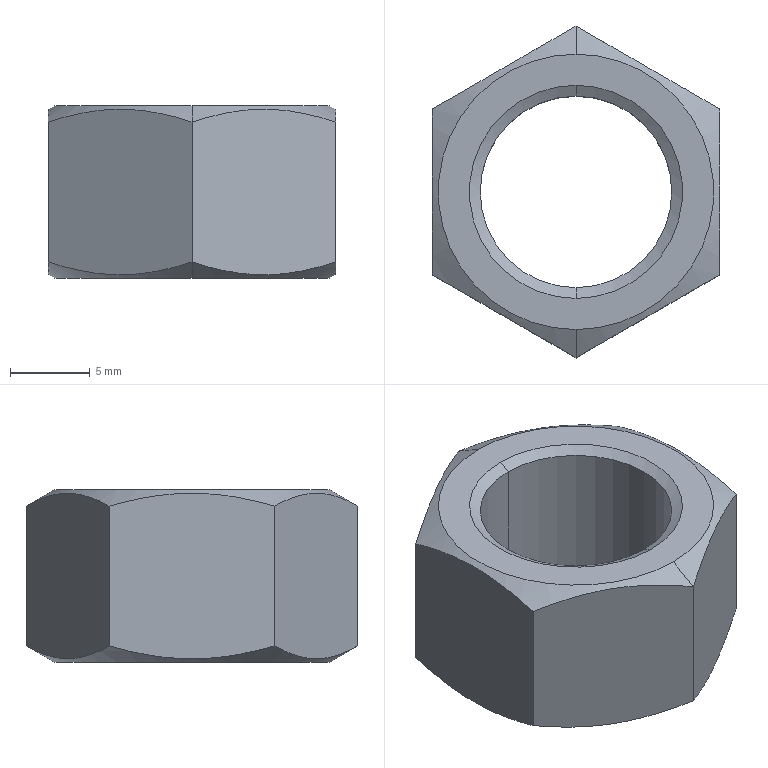Component | SolidWorks | Cylinder-1_hex nuts 1-fine pitch-grades ab gb-5 | 1 solid | 18 faces | box 18 x 20.78 x 10.8 mm | volume 1770 mm3 | cone 8 | plane 8 | cylinder 2 | commonest cylinder face diameters 12 x2
STEP:
#1=COLOUR_RGB('',0.7922,0.8196,0.9333);
#2=FILL_AREA_STYLE_COLOUR('',#1);
#3=FILL_AREA_STYLE('',(#2));
#4=SURFACE_STYLE_FILL_AREA(#3);
#5=SURFACE_SIDE_STYLE('',(#4));
#6=SURFACE_STYLE_USAGE(.BOTH.,#5);
#7=PRESENTATION_STYLE_ASSIGNMENT((#6));
#8=CARTESIAN_POINT('',(-8.211,1.906,-6.45));
#9=VERTEX_POINT('',#8);
#10=CARTESIAN_POINT('',(-8.211,2.378,-6.45));
#11=VERTEX_POINT('',#10);
#12=CARTESIAN_POINT('',(-8.211,2.142,-6.45));
#13=DIRECTION('',(-0.,0.,1.));
#14=DIRECTION('',(0.,-1.,0.));
#15=AXIS2_PLACEMENT_3D('',#12,#13,#14);
#16=CIRCLE('',#15,0.2362);
#17=EDGE_CURVE('',#9,#11,#16,.T.);
#18=ORIENTED_EDGE('',*,*,#17,.F.);
#19=CARTESIAN_POINT('',(-8.211,1.879,-6.435));
#20=VERTEX_POINT('',#19);
#21=CARTESIAN_POINT('',(-8.211,1.906,-6.45));
#22=DIRECTION('',(-0.,-0.866,0.5));
#23=VECTOR('',#22,39.37);
#24=LINE('',#21,#23);
#25=EDGE_CURVE('',#9,#20,#24,.T.);
#26=ORIENTED_EDGE('',*,*,#25,.T.);
#27=CARTESIAN_POINT('',(-8.211,2.405,-6.435));
#28=VERTEX_POINT('',#27);
#29=CARTESIAN_POINT('',(-8.211,2.142,-6.435));
#30=DIRECTION('',(0.,-0.,-1.));
#31=DIRECTION('',(0.,-1.,0.));
#32=AXIS2_PLACEMENT_3D('',#29,#30,#31);
#33=CIRCLE('',#32,0.2628);
#34=EDGE_CURVE('',#28,#20,#33,.T.);
#35=ORIENTED_EDGE('',*,*,#34,.F.);
#36=CARTESIAN_POINT('',(-8.211,2.378,-6.45));
#37=DIRECTION('',(0.,0.866,0.5));
#38=VECTOR('',#37,39.37);
#39=LINE('',#36,#38);
#40=EDGE_CURVE('',#11,#28,#39,.T.);
#41=ORIENTED_EDGE('',*,*,#40,.F.);
#42=EDGE_LOOP('',(#18,#26,#35,#41));
#43=FACE_OUTER_BOUND('',#42,.T.);
#44=CARTESIAN_POINT('',(-8.211,2.142,-6.45));
#45=DIRECTION('',(-0.,0.,1.));
#46=DIRECTION('',(0.,1.,0.));
#47=AXIS2_PLACEMENT_3D('',#44,#45,#46);
#48=CONICAL_SURFACE('',#47,0.2362,1.047);
#49=ADVANCED_FACE('',(#43),#48,.F.);
#50=CARTESIAN_POINT('',(-8.211,2.378,-6.834));
#51=VERTEX_POINT('',#50);
#52=CARTESIAN_POINT('',(-8.211,1.906,-6.834));
#53=VERTEX_POINT('',#52);
#54=CARTESIAN_POINT('',(-8.211,2.142,-6.834));
#55=DIRECTION('',(0.,-0.,-1.));
#56=DIRECTION('',(0.,-1.,0.));
#57=AXIS2_PLACEMENT_3D('',#54,#55,#56);
#58=CIRCLE('',#57,0.2362);
#59=EDGE_CURVE('',#51,#53,#58,.T.);
#60=ORIENTED_EDGE('',*,*,#59,.F.);
#61=CARTESIAN_POINT('',(-8.211,2.394,-6.86));
#62=VERTEX_POINT('',#61);
#63=CARTESIAN_POINT('',(-8.211,2.394,-6.86));
#64=DIRECTION('',(-0.,0.5,-0.866));
#65=VECTOR('',#64,39.37);
#66=LINE('',#63,#65);
#67=EDGE_CURVE('',#51,#62,#66,.T.);
#68=ORIENTED_EDGE('',*,*,#67,.T.);
#69=CARTESIAN_POINT('',(-8.211,1.891,-6.86));
#70=VERTEX_POINT('',#69);
#71=CARTESIAN_POINT('',(-8.211,2.142,-6.86));
#72=DIRECTION('',(-0.,0.,1.));
#73=DIRECTION('',(0.,-1.,0.));
#74=AXIS2_PLACEMENT_3D('',#71,#72,#73);
#75=CIRCLE('',#74,0.2516);
#76=EDGE_CURVE('',#70,#62,#75,.T.);
#77=ORIENTED_EDGE('',*,*,#76,.F.);
#78=CARTESIAN_POINT('',(-8.211,1.891,-6.86));
#79=DIRECTION('',(-0.,-0.5,-0.866));
#80=VECTOR('',#79,39.37);
#81=LINE('',#78,#80);
#82=EDGE_CURVE('',#53,#70,#81,.T.);
#83=ORIENTED_EDGE('',*,*,#82,.F.);
#84=EDGE_LOOP('',(#60,#68,#77,#83));
#85=FACE_OUTER_BOUND('',#84,.T.);
#86=CARTESIAN_POINT('',(-8.211,2.142,-6.86));
#87=DIRECTION('',(0.,-0.,-1.));
#88=DIRECTION('',(0.,-1.,0.));
#89=AXIS2_PLACEMENT_3D('',#86,#87,#88);
#90=CONICAL_SURFACE('',#89,0.2516,0.5236);
#91=ADVANCED_FACE('',(#85),#90,.F.);
#92=CARTESIAN_POINT('',(-8.211,1.803,-6.435));
#93=VERTEX_POINT('',#92);
#94=CARTESIAN_POINT('',(-8.211,2.482,-6.435));
#95=VERTEX_POINT('',#94);
#96=CARTESIAN_POINT('',(-8.211,2.142,-6.435));
#97=DIRECTION('',(0.,-0.,-1.));
#98=DIRECTION('',(0.,-1.,0.));
#99=AXIS2_PLACEMENT_3D('',#96,#97,#98);
#100=CIRCLE('',#99,0.3396);
#101=EDGE_CURVE('',#93,#95,#100,.T.);
#102=ORIENTED_EDGE('',*,*,#101,.T.);
#103=CARTESIAN_POINT('',(-8.211,2.551,-6.475));
#104=VERTEX_POINT('',#103);
#105=CARTESIAN_POINT('',(-8.211,2.482,-6.435));
#106=DIRECTION('',(-0.,0.866,-0.5));
#107=VECTOR('',#106,39.37);
#108=LINE('',#105,#107);
#109=EDGE_CURVE('',#95,#104,#108,.T.);
#110=ORIENTED_EDGE('',*,*,#109,.T.);
#111=CARTESIAN_POINT('',(-8.565,2.347,-6.475));
#112=VERTEX_POINT('',#111);
#113=CARTESIAN_POINT('',(-8.211,2.551,-6.475));
#114=CARTESIAN_POINT('',(-8.24,2.535,-6.466));
#115=CARTESIAN_POINT('',(-8.269,2.518,-6.458));
#116=CARTESIAN_POINT('',(-8.328,2.484,-6.447));
#117=CARTESIAN_POINT('',(-8.358,2.467,-6.444));
#118=CARTESIAN_POINT('',(-8.403,2.441,-6.444));
#119=CARTESIAN_POINT('',(-8.418,2.432,-6.444));
#120=CARTESIAN_POINT('',(-8.448,2.415,-6.447));
#121=CARTESIAN_POINT('',(-8.463,2.406,-6.449));
#122=CARTESIAN_POINT('',(-8.507,2.38,-6.458));
#123=CARTESIAN_POINT('',(-8.536,2.363,-6.466));
#124=CARTESIAN_POINT('',(-8.565,2.347,-6.475));
#125=B_SPLINE_CURVE_WITH_KNOTS('',3,(#113,#114,#115,#116,#117,#118,#119,#120,#121,#122,#123,#124),.UNSPECIFIED.,.F.,.F.,(4,2,2,2,2,4),(0.00000024,0.002624,0.005248,0.00656,0.007872,0.0105),.UNSPECIFIED.);
#126=EDGE_CURVE('',#104,#112,#125,.T.);
#127=ORIENTED_EDGE('',*,*,#126,.T.);
#128=CARTESIAN_POINT('',(-8.565,1.938,-6.475));
#129=VERTEX_POINT('',#128);
#130=CARTESIAN_POINT('',(-8.565,2.347,-6.475));
#131=CARTESIAN_POINT('',(-8.565,2.314,-6.466));
#132=CARTESIAN_POINT('',(-8.565,2.28,-6.458));
#133=CARTESIAN_POINT('',(-8.565,2.229,-6.449));
#134=CARTESIAN_POINT('',(-8.565,2.212,-6.447));
#135=CARTESIAN_POINT('',(-8.565,2.177,-6.444));
#136=CARTESIAN_POINT('',(-8.565,2.16,-6.444));
#137=CARTESIAN_POINT('',(-8.565,2.108,-6.444));
#138=CARTESIAN_POINT('',(-8.565,2.073,-6.447));
#139=CARTESIAN_POINT('',(-8.565,2.005,-6.458));
#140=CARTESIAN_POINT('',(-8.565,1.971,-6.466));
#141=CARTESIAN_POINT('',(-8.565,1.938,-6.475));
#142=B_SPLINE_CURVE_WITH_KNOTS('',3,(#130,#131,#132,#133,#134,#135,#136,#137,#138,#139,#140,#141),.UNSPECIFIED.,.F.,.F.,(4,2,2,2,2,4),(0.003845,0.006467,0.007778,0.009089,0.01171,0.01433),.UNSPECIFIED.);
#143=EDGE_CURVE('',#112,#129,#142,.T.);
#144=ORIENTED_EDGE('',*,*,#143,.T.);
#145=CARTESIAN_POINT('',(-8.211,1.733,-6.475));
#146=VERTEX_POINT('',#145);
#147=CARTESIAN_POINT('',(-8.565,1.938,-6.475));
#148=CARTESIAN_POINT('',(-8.536,1.921,-6.466));
#149=CARTESIAN_POINT('',(-8.507,1.904,-6.458));
#150=CARTESIAN_POINT('',(-8.448,1.87,-6.447));
#151=CARTESIAN_POINT('',(-8.419,1.853,-6.444));
#152=CARTESIAN_POINT('',(-8.373,1.827,-6.444));
#153=CARTESIAN_POINT('',(-8.358,1.818,-6.444));
#154=CARTESIAN_POINT('',(-8.328,1.801,-6.447));
#155=CARTESIAN_POINT('',(-8.313,1.792,-6.449));
#156=CARTESIAN_POINT('',(-8.269,1.767,-6.458));
#157=CARTESIAN_POINT('',(-8.24,1.75,-6.466));
#158=CARTESIAN_POINT('',(-8.211,1.733,-6.475));
#159=B_SPLINE_CURVE_WITH_KNOTS('',3,(#147,#148,#149,#150,#151,#152,#153,#154,#155,#156,#157,#158),.UNSPECIFIED.,.F.,.F.,(4,2,2,2,2,4),(0.00000024,0.002624,0.005248,0.00656,0.007872,0.0105),.UNSPECIFIED.);
#160=EDGE_CURVE('',#129,#146,#159,.T.);
#161=ORIENTED_EDGE('',*,*,#160,.T.);
#162=CARTESIAN_POINT('',(-8.211,1.803,-6.435));
#163=DIRECTION('',(-0.,-0.866,-0.5));
#164=VECTOR('',#163,39.37);
#165=LINE('',#162,#164);
#166=EDGE_CURVE('',#93,#146,#165,.T.);
#167=ORIENTED_EDGE('',*,*,#166,.F.);
#168=EDGE_LOOP('',(#102,#110,#127,#144,#161,#167));
#169=FACE_OUTER_BOUND('',#168,.T.);
#170=CARTESIAN_POINT('',(-8.211,2.142,-6.435));
#171=DIRECTION('',(0.,-0.,-1.));
#172=DIRECTION('',(0.,-1.,0.));
#173=AXIS2_PLACEMENT_3D('',#170,#171,#172);
#174=CONICAL_SURFACE('',#173,0.3396,1.047);
#175=ADVANCED_FACE('',(#169),#174,.T.);
#176=CARTESIAN_POINT('',(-8.211,1.803,-6.86));
#177=VERTEX_POINT('',#176);
#178=CARTESIAN_POINT('',(-8.211,2.482,-6.86));
#179=VERTEX_POINT('',#178);
#180=CARTESIAN_POINT('',(-8.211,2.142,-6.86));
#181=DIRECTION('',(0.,-0.,-1.));
#182=DIRECTION('',(0.,-1.,0.));
#183=AXIS2_PLACEMENT_3D('',#180,#181,#182);
#184=CIRCLE('',#183,0.3396);
#185=EDGE_CURVE('',#177,#179,#184,.T.);
#186=ORIENTED_EDGE('',*,*,#185,.F.);
#187=CARTESIAN_POINT('',(-8.211,1.733,-6.82));
#188=VERTEX_POINT('',#187);
#189=CARTESIAN_POINT('',(-8.211,1.733,-6.82));
#190=DIRECTION('',(-0.,-0.866,0.5));
#191=VECTOR('',#190,39.37);
#192=LINE('',#189,#191);
#193=EDGE_CURVE('',#177,#188,#192,.T.);
#194=ORIENTED_EDGE('',*,*,#193,.T.);
#195=CARTESIAN_POINT('',(-8.565,1.938,-6.82));
#196=VERTEX_POINT('',#195);
#197=CARTESIAN_POINT('',(-8.211,1.733,-6.82));
#198=CARTESIAN_POINT('',(-8.24,1.75,-6.83));
#199=CARTESIAN_POINT('',(-8.269,1.767,-6.838));
#200=CARTESIAN_POINT('',(-8.328,1.801,-6.849));
#201=CARTESIAN_POINT('',(-8.358,1.818,-6.852));
#202=CARTESIAN_POINT('',(-8.403,1.844,-6.852));
#203=CARTESIAN_POINT('',(-8.418,1.853,-6.851));
#204=CARTESIAN_POINT('',(-8.448,1.87,-6.848));
#205=CARTESIAN_POINT('',(-8.463,1.878,-6.846));
#206=CARTESIAN_POINT('',(-8.507,1.904,-6.838));
#207=CARTESIAN_POINT('',(-8.536,1.921,-6.83));
#208=CARTESIAN_POINT('',(-8.565,1.938,-6.82));
#209=B_SPLINE_CURVE_WITH_KNOTS('',3,(#197,#198,#199,#200,#201,#202,#203,#204,#205,#206,#207,#208),.UNSPECIFIED.,.F.,.F.,(4,2,2,2,2,4),(0.00000024,0.002624,0.005248,0.00656,0.007872,0.0105),.UNSPECIFIED.);
#210=EDGE_CURVE('',#188,#196,#209,.T.);
#211=ORIENTED_EDGE('',*,*,#210,.T.);
#212=CARTESIAN_POINT('',(-8.565,2.347,-6.82));
#213=VERTEX_POINT('',#212);
#214=CARTESIAN_POINT('',(-8.565,1.938,-6.82));
#215=CARTESIAN_POINT('',(-8.565,1.971,-6.83));
#216=CARTESIAN_POINT('',(-8.565,2.005,-6.838));
#217=CARTESIAN_POINT('',(-8.565,2.073,-6.849));
#218=CARTESIAN_POINT('',(-8.565,2.108,-6.852));
#219=CARTESIAN_POINT('',(-8.565,2.16,-6.852));
#220=CARTESIAN_POINT('',(-8.565,2.177,-6.851));
#221=CARTESIAN_POINT('',(-8.565,2.212,-6.848));
#222=CARTESIAN_POINT('',(-8.565,2.229,-6.846));
#223=CARTESIAN_POINT('',(-8.565,2.28,-6.838));
#224=CARTESIAN_POINT('',(-8.565,2.314,-6.83));
#225=CARTESIAN_POINT('',(-8.565,2.347,-6.82));
#226=B_SPLINE_CURVE_WITH_KNOTS('',3,(#214,#215,#216,#217,#218,#219,#220,#221,#222,#223,#224,#225),.UNSPECIFIED.,.F.,.F.,(4,2,2,2,2,4),(0.009237,0.01187,0.0145,0.01581,0.01712,0.01975),.UNSPECIFIED.);
#227=EDGE_CURVE('',#196,#213,#226,.T.);
#228=ORIENTED_EDGE('',*,*,#227,.T.);
#229=CARTESIAN_POINT('',(-8.211,2.551,-6.82));
#230=VERTEX_POINT('',#229);
#231=CARTESIAN_POINT('',(-8.565,2.347,-6.82));
#232=CARTESIAN_POINT('',(-8.536,2.363,-6.83));
#233=CARTESIAN_POINT('',(-8.507,2.38,-6.838));
#234=CARTESIAN_POINT('',(-8.448,2.414,-6.849));
#235=CARTESIAN_POINT('',(-8.419,2.431,-6.852));
#236=CARTESIAN_POINT('',(-8.373,2.458,-6.852));
#237=CARTESIAN_POINT('',(-8.358,2.466,-6.851));
#238=CARTESIAN_POINT('',(-8.328,2.484,-6.848));
#239=CARTESIAN_POINT('',(-8.313,2.492,-6.846));
#240=CARTESIAN_POINT('',(-8.269,2.518,-6.838));
#241=CARTESIAN_POINT('',(-8.24,2.535,-6.83));
#242=CARTESIAN_POINT('',(-8.211,2.551,-6.82));
#243=B_SPLINE_CURVE_WITH_KNOTS('',3,(#231,#232,#233,#234,#235,#236,#237,#238,#239,#240,#241,#242),.UNSPECIFIED.,.F.,.F.,(4,2,2,2,2,4),(0.00000024,0.002624,0.005248,0.00656,0.007872,0.0105),.UNSPECIFIED.);
#244=EDGE_CURVE('',#213,#230,#243,.T.);
#245=ORIENTED_EDGE('',*,*,#244,.T.);
#246=CARTESIAN_POINT('',(-8.211,2.551,-6.82));
#247=DIRECTION('',(0.,0.866,0.5));
#248=VECTOR('',#247,39.37);
#249=LINE('',#246,#248);
#250=EDGE_CURVE('',#179,#230,#249,.T.);
#251=ORIENTED_EDGE('',*,*,#250,.F.);
#252=EDGE_LOOP('',(#186,#194,#211,#228,#245,#251));
#253=FACE_OUTER_BOUND('',#252,.T.);
#254=CARTESIAN_POINT('',(-8.211,2.142,-6.82));
#255=DIRECTION('',(-0.,0.,1.));
#256=DIRECTION('',(0.,1.,0.));
#257=AXIS2_PLACEMENT_3D('',#254,#255,#256);
#258=CONICAL_SURFACE('',#257,0.4091,1.047);
#259=ADVANCED_FACE('',(#253),#258,.T.);
#260=ORIENTED_EDGE('',*,*,#59,.T.);
#261=CARTESIAN_POINT('',(-8.211,1.906,-6.86));
#262=DIRECTION('',(-0.,0.,1.));
#263=VECTOR('',#262,39.37);
#264=LINE('',#261,#263);
#265=EDGE_CURVE('',#53,#9,#264,.T.);
#266=ORIENTED_EDGE('',*,*,#265,.T.);
#267=ORIENTED_EDGE('',*,*,#17,.T.);
#268=CARTESIAN_POINT('',(-8.211,2.378,-6.86));
#269=DIRECTION('',(-0.,0.,1.));
#270=VECTOR('',#269,39.37);
#271=LINE('',#268,#270);
#272=EDGE_CURVE('',#51,#11,#271,.T.);
#273=ORIENTED_EDGE('',*,*,#272,.F.);
#274=EDGE_LOOP('',(#260,#266,#267,#273));
#275=FACE_OUTER_BOUND('',#274,.T.);
#276=CARTESIAN_POINT('',(-8.211,2.142,-6.86));
#277=DIRECTION('',(-0.,0.,1.));
#278=DIRECTION('',(0.,1.,0.));
#279=AXIS2_PLACEMENT_3D('',#276,#277,#278);
#280=CYLINDRICAL_SURFACE('',#279,0.2362);
#281=ADVANCED_FACE('',(#275),#280,.F.);
#282=CARTESIAN_POINT('',(-7.857,1.938,-6.475));
#283=VERTEX_POINT('',#282);
#284=CARTESIAN_POINT('',(-7.857,2.347,-6.475));
#285=VERTEX_POINT('',#284);
#286=CARTESIAN_POINT('',(-7.857,1.938,-6.475));
#287=CARTESIAN_POINT('',(-7.857,1.971,-6.466));
#288=CARTESIAN_POINT('',(-7.857,2.005,-6.458));
#289=CARTESIAN_POINT('',(-7.857,2.073,-6.447));
#290=CARTESIAN_POINT('',(-7.857,2.108,-6.444));
#291=CARTESIAN_POINT('',(-7.857,2.16,-6.444));
#292=CARTESIAN_POINT('',(-7.857,2.177,-6.444));
#293=CARTESIAN_POINT('',(-7.857,2.212,-6.447));
#294=CARTESIAN_POINT('',(-7.857,2.229,-6.449));
#295=CARTESIAN_POINT('',(-7.857,2.28,-6.458));
#296=CARTESIAN_POINT('',(-7.857,2.314,-6.466));
#297=CARTESIAN_POINT('',(-7.857,2.347,-6.475));
#298=B_SPLINE_CURVE_WITH_KNOTS('',3,(#286,#287,#288,#289,#290,#291,#292,#293,#294,#295,#296,#297),.UNSPECIFIED.,.F.,.F.,(4,2,2,2,2,4),(0.009237,0.01187,0.0145,0.01581,0.01712,0.01975),.UNSPECIFIED.);
#299=EDGE_CURVE('',#283,#285,#298,.T.);
#300=ORIENTED_EDGE('',*,*,#299,.F.);
#301=CARTESIAN_POINT('',(-7.857,1.938,-6.82));
#302=VERTEX_POINT('',#301);
#303=CARTESIAN_POINT('',(-7.857,1.938,-6.86));
#304=DIRECTION('',(-0.,0.,1.));
#305=VECTOR('',#304,39.37);
#306=LINE('',#303,#305);
#307=EDGE_CURVE('',#302,#283,#306,.T.);
#308=ORIENTED_EDGE('',*,*,#307,.F.);
#309=CARTESIAN_POINT('',(-7.857,2.347,-6.82));
#310=VERTEX_POINT('',#309);
#311=CARTESIAN_POINT('',(-7.857,2.347,-6.82));
#312=CARTESIAN_POINT('',(-7.857,2.314,-6.83));
#313=CARTESIAN_POINT('',(-7.857,2.28,-6.838));
#314=CARTESIAN_POINT('',(-7.857,2.229,-6.846));
#315=CARTESIAN_POINT('',(-7.857,2.212,-6.848));
#316=CARTESIAN_POINT('',(-7.857,2.177,-6.851));
#317=CARTESIAN_POINT('',(-7.857,2.16,-6.852));
#318=CARTESIAN_POINT('',(-7.857,2.108,-6.852));
#319=CARTESIAN_POINT('',(-7.857,2.073,-6.849));
#320=CARTESIAN_POINT('',(-7.857,2.005,-6.838));
#321=CARTESIAN_POINT('',(-7.857,1.971,-6.83));
#322=CARTESIAN_POINT('',(-7.857,1.938,-6.82));
#323=B_SPLINE_CURVE_WITH_KNOTS('',3,(#311,#312,#313,#314,#315,#316,#317,#318,#319,#320,#321,#322),.UNSPECIFIED.,.F.,.F.,(4,2,2,2,2,4),(0.003845,0.006467,0.007778,0.009089,0.01171,0.01433),.UNSPECIFIED.);
#324=EDGE_CURVE('',#310,#302,#323,.T.);
#325=ORIENTED_EDGE('',*,*,#324,.F.);
#326=CARTESIAN_POINT('',(-7.857,2.347,-6.86));
#327=DIRECTION('',(-0.,0.,1.));
#328=VECTOR('',#327,39.37);
#329=LINE('',#326,#328);
#330=EDGE_CURVE('',#310,#285,#329,.T.);
#331=ORIENTED_EDGE('',*,*,#330,.T.);
#332=EDGE_LOOP('',(#300,#308,#325,#331));
#333=FACE_OUTER_BOUND('',#332,.T.);
#334=CARTESIAN_POINT('',(-7.857,1.938,-6.86));
#335=DIRECTION('',(1.,-0.,0.));
#336=DIRECTION('',(0.,-0.,-1.));
#337=AXIS2_PLACEMENT_3D('',#334,#335,#336);
#338=PLANE('',#337);
#339=ADVANCED_FACE('',(#333),#338,.T.);
#340=CARTESIAN_POINT('',(-8.211,1.733,-6.475));
#341=CARTESIAN_POINT('',(-8.182,1.75,-6.466));
#342=CARTESIAN_POINT('',(-8.153,1.767,-6.458));
#343=CARTESIAN_POINT('',(-8.094,1.801,-6.447));
#344=CARTESIAN_POINT('',(-8.064,1.818,-6.444));
#345=CARTESIAN_POINT('',(-8.019,1.844,-6.444));
#346=CARTESIAN_POINT('',(-8.004,1.853,-6.444));
#347=CARTESIAN_POINT('',(-7.974,1.87,-6.447));
#348=CARTESIAN_POINT('',(-7.959,1.878,-6.449));
#349=CARTESIAN_POINT('',(-7.915,1.904,-6.458));
#350=CARTESIAN_POINT('',(-7.886,1.921,-6.466));
#351=CARTESIAN_POINT('',(-7.857,1.938,-6.475));
#352=B_SPLINE_CURVE_WITH_KNOTS('',3,(#340,#341,#342,#343,#344,#345,#346,#347,#348,#349,#350,#351),.UNSPECIFIED.,.F.,.F.,(4,2,2,2,2,4),(0.00000024,0.002624,0.005248,0.00656,0.007872,0.0105),.UNSPECIFIED.);
#353=EDGE_CURVE('',#146,#283,#352,.T.);
#354=ORIENTED_EDGE('',*,*,#353,.F.);
#355=CARTESIAN_POINT('',(-8.211,1.733,-6.86));
#356=DIRECTION('',(-0.,0.,1.));
#357=VECTOR('',#356,39.37);
#358=LINE('',#355,#357);
#359=EDGE_CURVE('',#188,#146,#358,.T.);
#360=ORIENTED_EDGE('',*,*,#359,.F.);
#361=CARTESIAN_POINT('',(-7.857,1.938,-6.82));
#362=CARTESIAN_POINT('',(-7.885,1.921,-6.83));
#363=CARTESIAN_POINT('',(-7.915,1.904,-6.838));
#364=CARTESIAN_POINT('',(-7.974,1.87,-6.849));
#365=CARTESIAN_POINT('',(-8.003,1.853,-6.852));
#366=CARTESIAN_POINT('',(-8.048,1.827,-6.852));
#367=CARTESIAN_POINT('',(-8.064,1.818,-6.851));
#368=CARTESIAN_POINT('',(-8.094,1.801,-6.848));
#369=CARTESIAN_POINT('',(-8.108,1.792,-6.846));
#370=CARTESIAN_POINT('',(-8.153,1.767,-6.838));
#371=CARTESIAN_POINT('',(-8.182,1.75,-6.83));
#372=CARTESIAN_POINT('',(-8.211,1.733,-6.82));
#373=B_SPLINE_CURVE_WITH_KNOTS('',3,(#361,#362,#363,#364,#365,#366,#367,#368,#369,#370,#371,#372),.UNSPECIFIED.,.F.,.F.,(4,2,2,2,2,4),(0.00000024,0.002624,0.005248,0.00656,0.007872,0.0105),.UNSPECIFIED.);
#374=EDGE_CURVE('',#302,#188,#373,.T.);
#375=ORIENTED_EDGE('',*,*,#374,.F.);
#376=ORIENTED_EDGE('',*,*,#307,.T.);
#377=EDGE_LOOP('',(#354,#360,#375,#376));
#378=FACE_OUTER_BOUND('',#377,.T.);
#379=CARTESIAN_POINT('',(-8.211,1.733,-6.86));
#380=DIRECTION('',(0.5,-0.866,0.));
#381=DIRECTION('',(0.866,0.5,-0.));
#382=AXIS2_PLACEMENT_3D('',#379,#380,#381);
#383=PLANE('',#382);
#384=ADVANCED_FACE('',(#378),#383,.T.);
#385=ORIENTED_EDGE('',*,*,#160,.F.);
#386=CARTESIAN_POINT('',(-8.565,1.938,-6.86));
#387=DIRECTION('',(-0.,0.,1.));
#388=VECTOR('',#387,39.37);
#389=LINE('',#386,#388);
#390=EDGE_CURVE('',#196,#129,#389,.T.);
#391=ORIENTED_EDGE('',*,*,#390,.F.);
#392=ORIENTED_EDGE('',*,*,#210,.F.);
#393=ORIENTED_EDGE('',*,*,#359,.T.);
#394=EDGE_LOOP('',(#385,#391,#392,#393));
#395=FACE_OUTER_BOUND('',#394,.T.);
#396=CARTESIAN_POINT('',(-8.565,1.938,-6.86));
#397=DIRECTION('',(-0.5,-0.866,0.));
#398=DIRECTION('',(0.866,-0.5,0.));
#399=AXIS2_PLACEMENT_3D('',#396,#397,#398);
#400=PLANE('',#399);
#401=ADVANCED_FACE('',(#395),#400,.T.);
#402=ORIENTED_EDGE('',*,*,#143,.F.);
#403=CARTESIAN_POINT('',(-8.565,2.347,-6.86));
#404=DIRECTION('',(-0.,0.,1.));
#405=VECTOR('',#404,39.37);
#406=LINE('',#403,#405);
#407=EDGE_CURVE('',#213,#112,#406,.T.);
#408=ORIENTED_EDGE('',*,*,#407,.F.);
#409=ORIENTED_EDGE('',*,*,#227,.F.);
#410=ORIENTED_EDGE('',*,*,#390,.T.);
#411=EDGE_LOOP('',(#402,#408,#409,#410));
#412=FACE_OUTER_BOUND('',#411,.T.);
#413=CARTESIAN_POINT('',(-8.565,2.347,-6.86));
#414=DIRECTION('',(-1.,0.,-0.));
#415=DIRECTION('',(-0.,-1.,0.));
#416=AXIS2_PLACEMENT_3D('',#413,#414,#415);
#417=PLANE('',#416);
#418=ADVANCED_FACE('',(#412),#417,.T.);
#419=ORIENTED_EDGE('',*,*,#126,.F.);
#420=CARTESIAN_POINT('',(-8.211,2.551,-6.86));
#421=DIRECTION('',(-0.,0.,1.));
#422=VECTOR('',#421,39.37);
#423=LINE('',#420,#422);
#424=EDGE_CURVE('',#230,#104,#423,.T.);
#425=ORIENTED_EDGE('',*,*,#424,.F.);
#426=ORIENTED_EDGE('',*,*,#244,.F.);
#427=ORIENTED_EDGE('',*,*,#407,.T.);
#428=EDGE_LOOP('',(#419,#425,#426,#427));
#429=FACE_OUTER_BOUND('',#428,.T.);
#430=CARTESIAN_POINT('',(-8.211,2.551,-6.86));
#431=DIRECTION('',(-0.5,0.866,-0.));
#432=DIRECTION('',(-0.866,-0.5,0.));
#433=AXIS2_PLACEMENT_3D('',#430,#431,#432);
#434=PLANE('',#433);
#435=ADVANCED_FACE('',(#429),#434,.T.);
#436=CARTESIAN_POINT('',(-7.857,2.347,-6.475));
#437=CARTESIAN_POINT('',(-7.885,2.363,-6.466));
#438=CARTESIAN_POINT('',(-7.915,2.38,-6.458));
#439=CARTESIAN_POINT('',(-7.974,2.414,-6.447));
#440=CARTESIAN_POINT('',(-8.003,2.431,-6.444));
#441=CARTESIAN_POINT('',(-8.048,2.458,-6.444));
#442=CARTESIAN_POINT('',(-8.064,2.466,-6.444));
#443=CARTESIAN_POINT('',(-8.094,2.484,-6.447));
#444=CARTESIAN_POINT('',(-8.108,2.492,-6.449));
#445=CARTESIAN_POINT('',(-8.153,2.518,-6.458));
#446=CARTESIAN_POINT('',(-8.182,2.535,-6.466));
#447=CARTESIAN_POINT('',(-8.211,2.551,-6.475));
#448=B_SPLINE_CURVE_WITH_KNOTS('',3,(#436,#437,#438,#439,#440,#441,#442,#443,#444,#445,#446,#447),.UNSPECIFIED.,.F.,.F.,(4,2,2,2,2,4),(0.00000024,0.002624,0.005248,0.00656,0.007872,0.0105),.UNSPECIFIED.);
#449=EDGE_CURVE('',#285,#104,#448,.T.);
#450=ORIENTED_EDGE('',*,*,#449,.F.);
#451=ORIENTED_EDGE('',*,*,#330,.F.);
#452=CARTESIAN_POINT('',(-8.211,2.551,-6.82));
#453=CARTESIAN_POINT('',(-8.182,2.535,-6.83));
#454=CARTESIAN_POINT('',(-8.153,2.518,-6.838));
#455=CARTESIAN_POINT('',(-8.094,2.484,-6.849));
#456=CARTESIAN_POINT('',(-8.064,2.467,-6.852));
#457=CARTESIAN_POINT('',(-8.019,2.441,-6.852));
#458=CARTESIAN_POINT('',(-8.004,2.432,-6.851));
#459=CARTESIAN_POINT('',(-7.974,2.415,-6.848));
#460=CARTESIAN_POINT('',(-7.959,2.406,-6.846));
#461=CARTESIAN_POINT('',(-7.915,2.38,-6.838));
#462=CARTESIAN_POINT('',(-7.886,2.363,-6.83));
#463=CARTESIAN_POINT('',(-7.857,2.347,-6.82));
#464=B_SPLINE_CURVE_WITH_KNOTS('',3,(#452,#453,#454,#455,#456,#457,#458,#459,#460,#461,#462,#463),.UNSPECIFIED.,.F.,.F.,(4,2,2,2,2,4),(0.00000024,0.002624,0.005248,0.00656,0.007872,0.0105),.UNSPECIFIED.);
#465=EDGE_CURVE('',#230,#310,#464,.T.);
#466=ORIENTED_EDGE('',*,*,#465,.F.);
#467=ORIENTED_EDGE('',*,*,#424,.T.);
#468=EDGE_LOOP('',(#450,#451,#466,#467));
#469=FACE_OUTER_BOUND('',#468,.T.);
#470=CARTESIAN_POINT('',(-7.857,2.347,-6.86));
#471=DIRECTION('',(0.5,0.866,-0.));
#472=DIRECTION('',(-0.866,0.5,-0.));
#473=AXIS2_PLACEMENT_3D('',#470,#471,#472);
#474=PLANE('',#473);
#475=ADVANCED_FACE('',(#469),#474,.T.);
#476=ORIENTED_EDGE('',*,*,#76,.T.);
#477=CARTESIAN_POINT('',(-8.211,2.142,-6.86));
#478=DIRECTION('',(-0.,0.,1.));
#479=DIRECTION('',(0.,-1.,0.));
#480=AXIS2_PLACEMENT_3D('',#477,#478,#479);
#481=CIRCLE('',#480,0.2516);
#482=EDGE_CURVE('',#62,#70,#481,.T.);
#483=ORIENTED_EDGE('',*,*,#482,.T.);
#484=EDGE_LOOP('',(#476,#483));
#485=FACE_BOUND('',#484,.T.);
#486=CARTESIAN_POINT('',(-8.211,2.142,-6.86));
#487=DIRECTION('',(0.,-0.,-1.));
#488=DIRECTION('',(0.,-1.,0.));
#489=AXIS2_PLACEMENT_3D('',#486,#487,#488);
#490=CIRCLE('',#489,0.3396);
#491=EDGE_CURVE('',#179,#177,#490,.T.);
#492=ORIENTED_EDGE('',*,*,#491,.T.);
#493=ORIENTED_EDGE('',*,*,#185,.T.);
#494=EDGE_LOOP('',(#492,#493));
#495=FACE_OUTER_BOUND('',#494,.T.);
#496=CARTESIAN_POINT('',(-7.857,1.528,-6.86));
#497=DIRECTION('',(0.,-0.,-1.));
#498=DIRECTION('',(-0.,-1.,0.));
#499=AXIS2_PLACEMENT_3D('',#496,#497,#498);
#500=PLANE('',#499);
#501=ADVANCED_FACE('',(#485,#495),#500,.T.);
#502=ORIENTED_EDGE('',*,*,#34,.T.);
#503=CARTESIAN_POINT('',(-8.211,2.142,-6.435));
#504=DIRECTION('',(0.,-0.,-1.));
#505=DIRECTION('',(0.,-1.,0.));
#506=AXIS2_PLACEMENT_3D('',#503,#504,#505);
#507=CIRCLE('',#506,0.2628);
#508=EDGE_CURVE('',#20,#28,#507,.T.);
#509=ORIENTED_EDGE('',*,*,#508,.T.);
#510=EDGE_LOOP('',(#502,#509));
#511=FACE_BOUND('',#510,.T.);
#512=ORIENTED_EDGE('',*,*,#101,.F.);
#513=CARTESIAN_POINT('',(-8.211,2.142,-6.435));
#514=DIRECTION('',(0.,-0.,-1.));
#515=DIRECTION('',(0.,-1.,0.));
#516=AXIS2_PLACEMENT_3D('',#513,#514,#515);
#517=CIRCLE('',#516,0.3396);
#518=EDGE_CURVE('',#95,#93,#517,.T.);
#519=ORIENTED_EDGE('',*,*,#518,.F.);
#520=EDGE_LOOP('',(#512,#519));
#521=FACE_OUTER_BOUND('',#520,.T.);
#522=CARTESIAN_POINT('',(-7.857,1.528,-6.435));
#523=DIRECTION('',(0.,-0.,-1.));
#524=DIRECTION('',(-0.,-1.,0.));
#525=AXIS2_PLACEMENT_3D('',#522,#523,#524);
#526=PLANE('',#525);
#527=ADVANCED_FACE('',(#511,#521),#526,.F.);
#528=ORIENTED_EDGE('',*,*,#265,.F.);
#529=CARTESIAN_POINT('',(-8.211,2.142,-6.834));
#530=DIRECTION('',(0.,-0.,-1.));
#531=DIRECTION('',(0.,-1.,0.));
#532=AXIS2_PLACEMENT_3D('',#529,#530,#531);
#533=CIRCLE('',#532,0.2362);
#534=EDGE_CURVE('',#53,#51,#533,.T.);
#535=ORIENTED_EDGE('',*,*,#534,.T.);
#536=ORIENTED_EDGE('',*,*,#272,.T.);
#537=CARTESIAN_POINT('',(-8.211,2.142,-6.45));
#538=DIRECTION('',(-0.,0.,1.));
#539=DIRECTION('',(0.,-1.,0.));
#540=AXIS2_PLACEMENT_3D('',#537,#538,#539);
#541=CIRCLE('',#540,0.2362);
#542=EDGE_CURVE('',#11,#9,#541,.T.);
#543=ORIENTED_EDGE('',*,*,#542,.T.);
#544=EDGE_LOOP('',(#528,#535,#536,#543));
#545=FACE_OUTER_BOUND('',#544,.T.);
#546=CARTESIAN_POINT('',(-8.211,2.142,-6.86));
#547=DIRECTION('',(-0.,0.,1.));
#548=DIRECTION('',(0.,1.,0.));
#549=AXIS2_PLACEMENT_3D('',#546,#547,#548);
#550=CYLINDRICAL_SURFACE('',#549,0.2362);
#551=ADVANCED_FACE('',(#545),#550,.F.);
#552=ORIENTED_EDGE('',*,*,#193,.F.);
#553=ORIENTED_EDGE('',*,*,#491,.F.);
#554=ORIENTED_EDGE('',*,*,#250,.T.);
#555=ORIENTED_EDGE('',*,*,#465,.T.);
#556=ORIENTED_EDGE('',*,*,#324,.T.);
#557=ORIENTED_EDGE('',*,*,#374,.T.);
#558=EDGE_LOOP('',(#552,#553,#554,#555,#556,#557));
#559=FACE_OUTER_BOUND('',#558,.T.);
#560=CARTESIAN_POINT('',(-8.211,2.142,-6.82));
#561=DIRECTION('',(-0.,0.,1.));
#562=DIRECTION('',(0.,1.,0.));
#563=AXIS2_PLACEMENT_3D('',#560,#561,#562);
#564=CONICAL_SURFACE('',#563,0.4091,1.047);
#565=ADVANCED_FACE('',(#559),#564,.T.);
#566=ORIENTED_EDGE('',*,*,#109,.F.);
#567=ORIENTED_EDGE('',*,*,#518,.T.);
#568=ORIENTED_EDGE('',*,*,#166,.T.);
#569=ORIENTED_EDGE('',*,*,#353,.T.);
#570=ORIENTED_EDGE('',*,*,#299,.T.);
#571=ORIENTED_EDGE('',*,*,#449,.T.);
#572=EDGE_LOOP('',(#566,#567,#568,#569,#570,#571));
#573=FACE_OUTER_BOUND('',#572,.T.);
#574=CARTESIAN_POINT('',(-8.211,2.142,-6.435));
#575=DIRECTION('',(0.,-0.,-1.));
#576=DIRECTION('',(0.,-1.,0.));
#577=AXIS2_PLACEMENT_3D('',#574,#575,#576);
#578=CONICAL_SURFACE('',#577,0.3396,1.047);
#579=ADVANCED_FACE('',(#573),#578,.T.);
#580=ORIENTED_EDGE('',*,*,#67,.F.);
#581=ORIENTED_EDGE('',*,*,#534,.F.);
#582=ORIENTED_EDGE('',*,*,#82,.T.);
#583=ORIENTED_EDGE('',*,*,#482,.F.);
#584=EDGE_LOOP('',(#580,#581,#582,#583));
#585=FACE_OUTER_BOUND('',#584,.T.);
#586=CARTESIAN_POINT('',(-8.211,2.142,-6.86));
#587=DIRECTION('',(0.,-0.,-1.));
#588=DIRECTION('',(0.,-1.,0.));
#589=AXIS2_PLACEMENT_3D('',#586,#587,#588);
#590=CONICAL_SURFACE('',#589,0.2516,0.5236);
#591=ADVANCED_FACE('',(#585),#590,.F.);
#592=ORIENTED_EDGE('',*,*,#25,.F.);
#593=ORIENTED_EDGE('',*,*,#542,.F.);
#594=ORIENTED_EDGE('',*,*,#40,.T.);
#595=ORIENTED_EDGE('',*,*,#508,.F.);
#596=EDGE_LOOP('',(#592,#593,#594,#595));
#597=FACE_OUTER_BOUND('',#596,.T.);
#598=CARTESIAN_POINT('',(-8.211,2.142,-6.45));
#599=DIRECTION('',(-0.,0.,1.));
#600=DIRECTION('',(0.,1.,0.));
#601=AXIS2_PLACEMENT_3D('',#598,#599,#600);
#602=CONICAL_SURFACE('',#601,0.2362,1.047);
#603=ADVANCED_FACE('',(#597),#602,.F.);
#604=CLOSED_SHELL('',(#49,#91,#175,#259,#281,#339,#384,#401,#418,#435,#475,#501,#527,#551,#565,#579,#591,#603));
#605=MANIFOLD_SOLID_BREP('',#604);
#606=STYLED_ITEM('',(#7),#605);
#607=PRESENTATION_LAYER_ASSIGNMENT('','',(#606));
#608=CARTESIAN_POINT('',(0.,0.,0.));
#609=DIRECTION('',(0.,0.,1.));
#610=DIRECTION('',(1.,0.,0.));
#611=AXIS2_PLACEMENT_3D('',#608,#609,#610);
#612=(LENGTH_UNIT()NAMED_UNIT(*)SI_UNIT($,.METRE.));
#613=LENGTH_MEASURE_WITH_UNIT(LENGTH_MEASURE(0.0254),#612);
#614=DIMENSIONAL_EXPONENTS(1.,0.,0.,0.,0.,0.,0.);
#615=(CONVERSION_BASED_UNIT('',#613)LENGTH_UNIT()NAMED_UNIT(#614));
#616=UNCERTAINTY_MEASURE_WITH_UNIT(LENGTH_MEASURE(0.00001),#615,'','');
#617=(NAMED_UNIT(*)PLANE_ANGLE_UNIT()SI_UNIT($,.RADIAN.));
#618=(NAMED_UNIT(*)SI_UNIT($,.STERADIAN.)SOLID_ANGLE_UNIT());
#619=(GEOMETRIC_REPRESENTATION_CONTEXT(3)GLOBAL_UNCERTAINTY_ASSIGNED_CONTEXT((#616))GLOBAL_UNIT_ASSIGNED_CONTEXT((#615,#617,#618))REPRESENTATION_CONTEXT('',''));
#620=ADVANCED_BREP_SHAPE_REPRESENTATION('',(#605,#611),#619);
#621=(LENGTH_UNIT()NAMED_UNIT(*)SI_UNIT($,.METRE.));
#622=LENGTH_MEASURE_WITH_UNIT(LENGTH_MEASURE(0.0254),#621);
#623=DIMENSIONAL_EXPONENTS(1.,0.,0.,0.,0.,0.,0.);
#624=(CONVERSION_BASED_UNIT('',#622)LENGTH_UNIT()NAMED_UNIT(#623));
#625=UNCERTAINTY_MEASURE_WITH_UNIT(LENGTH_MEASURE(0.00001),#624,'','');
#626=(NAMED_UNIT(*)PLANE_ANGLE_UNIT()SI_UNIT($,.RADIAN.));
#627=(NAMED_UNIT(*)SI_UNIT($,.STERADIAN.)SOLID_ANGLE_UNIT());
#628=(GEOMETRIC_REPRESENTATION_CONTEXT(3)GLOBAL_UNCERTAINTY_ASSIGNED_CONTEXT((#625))GLOBAL_UNIT_ASSIGNED_CONTEXT((#624,#626,#627))REPRESENTATION_CONTEXT('',''));
#629=MECHANICAL_DESIGN_GEOMETRIC_PRESENTATION_REPRESENTATION('',(#606),#628);